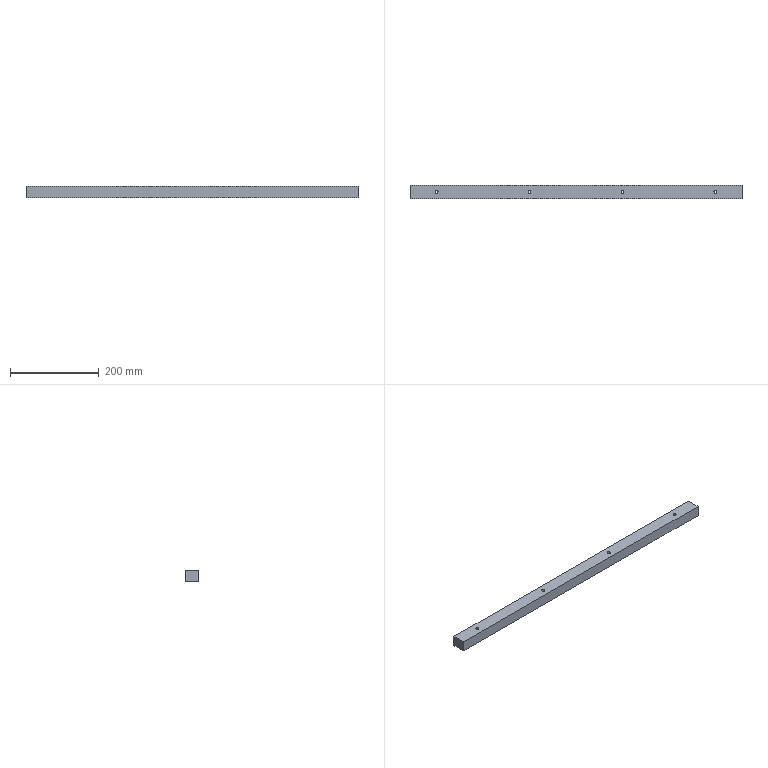Component | SolidWorks | DC-Motor-112-1 | 1 solid | 26 faces | box 750 x 30 x 25 mm | volume 557522 mm3 | cylinder 16 | plane 10 | commonest cylinder face diameters 11 x8 6.6 x8
build123d program:
from build123d import *

# Parameters (mm, degrees)
SKETCH1_W                                       = 750
SKETCH1_H                                       = 30
BOSS_EXTRUDE1_DEPTH                             = 12.5
M6_HEX_SOCKET_HEAD_CAP_SCREW_CBORE1_D           = 6.6
M6_HEX_SOCKET_HEAD_CAP_SCREW_CBORE1_CBORE_D     = 11
M6_HEX_SOCKET_HEAD_CAP_SCREW_CBORE1_CBORE_DEPTH = 6.4


with BuildPart() as part:
    # Sketch1 → Boss-Extrude1 (new, symmetric)
    with BuildSketch(Plane.XY):
        Rectangle(SKETCH1_W, SKETCH1_H)
    extrude(amount=BOSS_EXTRUDE1_DEPTH, both=True)

    # M6 Hex Socket Head Cap Screw CBORE1 (through all)
    with Locations(Plane.XY.offset(12.5)):
        with Locations((-315, 0), (-105, 0), (105, 0), (315, 0)):
            CounterBoreHole(M6_HEX_SOCKET_HEAD_CAP_SCREW_CBORE1_D / 2, M6_HEX_SOCKET_HEAD_CAP_SCREW_CBORE1_CBORE_D / 2, M6_HEX_SOCKET_HEAD_CAP_SCREW_CBORE1_CBORE_DEPTH)


solid = part.part

# Placed as in the assembly
solid = solid.moved(Location((177.208, 371.801, -438.5), (180, 0, 0)))
STEP:
#1=COLOUR_RGB('',0.7922,0.8196,0.9333);
#2=FILL_AREA_STYLE_COLOUR('',#1);
#3=FILL_AREA_STYLE('',(#2));
#4=SURFACE_STYLE_FILL_AREA(#3);
#5=SURFACE_SIDE_STYLE('',(#4));
#6=SURFACE_STYLE_USAGE(.BOTH.,#5);
#7=PRESENTATION_STYLE_ASSIGNMENT((#6));
#8=CARTESIAN_POINT('',(19.595,14.638,-17.504));
#9=VERTEX_POINT('',#8);
#10=CARTESIAN_POINT('',(19.162,14.638,-17.504));
#11=VERTEX_POINT('',#10);
#12=CARTESIAN_POINT('',(19.378,14.638,-17.504));
#13=DIRECTION('',(0.,0.,-1.));
#14=DIRECTION('',(-1.,0.,0.));
#15=AXIS2_PLACEMENT_3D('',#12,#13,#14);
#16=CIRCLE('',#15,0.2165);
#17=EDGE_CURVE('',#9,#11,#16,.T.);
#18=ORIENTED_EDGE('',*,*,#17,.F.);
#19=CARTESIAN_POINT('',(19.595,14.638,-17.756));
#20=VERTEX_POINT('',#19);
#21=CARTESIAN_POINT('',(19.595,14.638,-17.756));
#22=DIRECTION('',(0.,0.,-1.));
#23=VECTOR('',#22,39.37);
#24=LINE('',#21,#23);
#25=EDGE_CURVE('',#9,#20,#24,.T.);
#26=ORIENTED_EDGE('',*,*,#25,.T.);
#27=CARTESIAN_POINT('',(19.162,14.638,-17.756));
#28=VERTEX_POINT('',#27);
#29=CARTESIAN_POINT('',(19.378,14.638,-17.756));
#30=DIRECTION('',(0.,0.,-1.));
#31=DIRECTION('',(-1.,0.,0.));
#32=AXIS2_PLACEMENT_3D('',#29,#30,#31);
#33=CIRCLE('',#32,0.2165);
#34=EDGE_CURVE('',#20,#28,#33,.T.);
#35=ORIENTED_EDGE('',*,*,#34,.T.);
#36=CARTESIAN_POINT('',(19.162,14.638,-17.756));
#37=DIRECTION('',(0.,0.,-1.));
#38=VECTOR('',#37,39.37);
#39=LINE('',#36,#38);
#40=EDGE_CURVE('',#11,#28,#39,.T.);
#41=ORIENTED_EDGE('',*,*,#40,.F.);
#42=EDGE_LOOP('',(#18,#26,#35,#41));
#43=FACE_OUTER_BOUND('',#42,.T.);
#44=CARTESIAN_POINT('',(19.378,14.638,-17.756));
#45=DIRECTION('',(0.,0.,-1.));
#46=DIRECTION('',(-1.,0.,0.));
#47=AXIS2_PLACEMENT_3D('',#44,#45,#46);
#48=CYLINDRICAL_SURFACE('',#47,0.2165);
#49=ADVANCED_FACE('',(#43),#48,.F.);
#50=CARTESIAN_POINT('',(19.508,14.638,-16.772));
#51=VERTEX_POINT('',#50);
#52=CARTESIAN_POINT('',(19.248,14.638,-16.772));
#53=VERTEX_POINT('',#52);
#54=CARTESIAN_POINT('',(19.378,14.638,-16.772));
#55=DIRECTION('',(0.,0.,-1.));
#56=DIRECTION('',(-1.,0.,0.));
#57=AXIS2_PLACEMENT_3D('',#54,#55,#56);
#58=CIRCLE('',#57,0.1299);
#59=EDGE_CURVE('',#51,#53,#58,.T.);
#60=ORIENTED_EDGE('',*,*,#59,.F.);
#61=CARTESIAN_POINT('',(19.508,14.638,-17.504));
#62=VERTEX_POINT('',#61);
#63=CARTESIAN_POINT('',(19.508,14.638,-17.756));
#64=DIRECTION('',(0.,0.,-1.));
#65=VECTOR('',#64,39.37);
#66=LINE('',#63,#65);
#67=EDGE_CURVE('',#51,#62,#66,.T.);
#68=ORIENTED_EDGE('',*,*,#67,.T.);
#69=CARTESIAN_POINT('',(19.248,14.638,-17.504));
#70=VERTEX_POINT('',#69);
#71=CARTESIAN_POINT('',(19.378,14.638,-17.504));
#72=DIRECTION('',(0.,0.,-1.));
#73=DIRECTION('',(-1.,0.,0.));
#74=AXIS2_PLACEMENT_3D('',#71,#72,#73);
#75=CIRCLE('',#74,0.1299);
#76=EDGE_CURVE('',#62,#70,#75,.T.);
#77=ORIENTED_EDGE('',*,*,#76,.T.);
#78=CARTESIAN_POINT('',(19.248,14.638,-17.756));
#79=DIRECTION('',(0.,0.,-1.));
#80=VECTOR('',#79,39.37);
#81=LINE('',#78,#80);
#82=EDGE_CURVE('',#53,#70,#81,.T.);
#83=ORIENTED_EDGE('',*,*,#82,.F.);
#84=EDGE_LOOP('',(#60,#68,#77,#83));
#85=FACE_OUTER_BOUND('',#84,.T.);
#86=CARTESIAN_POINT('',(19.378,14.638,-17.756));
#87=DIRECTION('',(0.,0.,-1.));
#88=DIRECTION('',(-1.,0.,0.));
#89=AXIS2_PLACEMENT_3D('',#86,#87,#88);
#90=CYLINDRICAL_SURFACE('',#89,0.1299);
#91=ADVANCED_FACE('',(#85),#90,.F.);
#92=CARTESIAN_POINT('',(11.327,14.638,-17.504));
#93=VERTEX_POINT('',#92);
#94=CARTESIAN_POINT('',(10.894,14.638,-17.504));
#95=VERTEX_POINT('',#94);
#96=CARTESIAN_POINT('',(11.111,14.638,-17.504));
#97=DIRECTION('',(0.,0.,-1.));
#98=DIRECTION('',(-1.,0.,0.));
#99=AXIS2_PLACEMENT_3D('',#96,#97,#98);
#100=CIRCLE('',#99,0.2165);
#101=EDGE_CURVE('',#93,#95,#100,.T.);
#102=ORIENTED_EDGE('',*,*,#101,.F.);
#103=CARTESIAN_POINT('',(11.327,14.638,-17.756));
#104=VERTEX_POINT('',#103);
#105=CARTESIAN_POINT('',(11.327,14.638,-17.756));
#106=DIRECTION('',(0.,0.,-1.));
#107=VECTOR('',#106,39.37);
#108=LINE('',#105,#107);
#109=EDGE_CURVE('',#93,#104,#108,.T.);
#110=ORIENTED_EDGE('',*,*,#109,.T.);
#111=CARTESIAN_POINT('',(10.894,14.638,-17.756));
#112=VERTEX_POINT('',#111);
#113=CARTESIAN_POINT('',(11.111,14.638,-17.756));
#114=DIRECTION('',(0.,0.,-1.));
#115=DIRECTION('',(-1.,0.,0.));
#116=AXIS2_PLACEMENT_3D('',#113,#114,#115);
#117=CIRCLE('',#116,0.2165);
#118=EDGE_CURVE('',#104,#112,#117,.T.);
#119=ORIENTED_EDGE('',*,*,#118,.T.);
#120=CARTESIAN_POINT('',(10.894,14.638,-17.756));
#121=DIRECTION('',(0.,0.,-1.));
#122=VECTOR('',#121,39.37);
#123=LINE('',#120,#122);
#124=EDGE_CURVE('',#95,#112,#123,.T.);
#125=ORIENTED_EDGE('',*,*,#124,.F.);
#126=EDGE_LOOP('',(#102,#110,#119,#125));
#127=FACE_OUTER_BOUND('',#126,.T.);
#128=CARTESIAN_POINT('',(11.111,14.638,-17.756));
#129=DIRECTION('',(0.,0.,-1.));
#130=DIRECTION('',(-1.,0.,0.));
#131=AXIS2_PLACEMENT_3D('',#128,#129,#130);
#132=CYLINDRICAL_SURFACE('',#131,0.2165);
#133=ADVANCED_FACE('',(#127),#132,.F.);
#134=CARTESIAN_POINT('',(11.24,14.638,-16.772));
#135=VERTEX_POINT('',#134);
#136=CARTESIAN_POINT('',(10.981,14.638,-16.772));
#137=VERTEX_POINT('',#136);
#138=CARTESIAN_POINT('',(11.111,14.638,-16.772));
#139=DIRECTION('',(0.,0.,-1.));
#140=DIRECTION('',(-1.,0.,0.));
#141=AXIS2_PLACEMENT_3D('',#138,#139,#140);
#142=CIRCLE('',#141,0.1299);
#143=EDGE_CURVE('',#135,#137,#142,.T.);
#144=ORIENTED_EDGE('',*,*,#143,.F.);
#145=CARTESIAN_POINT('',(11.24,14.638,-17.504));
#146=VERTEX_POINT('',#145);
#147=CARTESIAN_POINT('',(11.24,14.638,-17.756));
#148=DIRECTION('',(0.,0.,-1.));
#149=VECTOR('',#148,39.37);
#150=LINE('',#147,#149);
#151=EDGE_CURVE('',#135,#146,#150,.T.);
#152=ORIENTED_EDGE('',*,*,#151,.T.);
#153=CARTESIAN_POINT('',(10.981,14.638,-17.504));
#154=VERTEX_POINT('',#153);
#155=CARTESIAN_POINT('',(11.111,14.638,-17.504));
#156=DIRECTION('',(0.,0.,-1.));
#157=DIRECTION('',(-1.,0.,0.));
#158=AXIS2_PLACEMENT_3D('',#155,#156,#157);
#159=CIRCLE('',#158,0.1299);
#160=EDGE_CURVE('',#146,#154,#159,.T.);
#161=ORIENTED_EDGE('',*,*,#160,.T.);
#162=CARTESIAN_POINT('',(10.981,14.638,-17.756));
#163=DIRECTION('',(0.,0.,-1.));
#164=VECTOR('',#163,39.37);
#165=LINE('',#162,#164);
#166=EDGE_CURVE('',#137,#154,#165,.T.);
#167=ORIENTED_EDGE('',*,*,#166,.F.);
#168=EDGE_LOOP('',(#144,#152,#161,#167));
#169=FACE_OUTER_BOUND('',#168,.T.);
#170=CARTESIAN_POINT('',(11.111,14.638,-17.756));
#171=DIRECTION('',(0.,0.,-1.));
#172=DIRECTION('',(-1.,0.,0.));
#173=AXIS2_PLACEMENT_3D('',#170,#171,#172);
#174=CYLINDRICAL_SURFACE('',#173,0.1299);
#175=ADVANCED_FACE('',(#169),#174,.F.);
#176=CARTESIAN_POINT('',(3.059,14.638,-17.504));
#177=VERTEX_POINT('',#176);
#178=CARTESIAN_POINT('',(2.626,14.638,-17.504));
#179=VERTEX_POINT('',#178);
#180=CARTESIAN_POINT('',(2.843,14.638,-17.504));
#181=DIRECTION('',(0.,0.,-1.));
#182=DIRECTION('',(-1.,0.,0.));
#183=AXIS2_PLACEMENT_3D('',#180,#181,#182);
#184=CIRCLE('',#183,0.2165);
#185=EDGE_CURVE('',#177,#179,#184,.T.);
#186=ORIENTED_EDGE('',*,*,#185,.F.);
#187=CARTESIAN_POINT('',(3.059,14.638,-17.756));
#188=VERTEX_POINT('',#187);
#189=CARTESIAN_POINT('',(3.059,14.638,-17.756));
#190=DIRECTION('',(0.,0.,-1.));
#191=VECTOR('',#190,39.37);
#192=LINE('',#189,#191);
#193=EDGE_CURVE('',#177,#188,#192,.T.);
#194=ORIENTED_EDGE('',*,*,#193,.T.);
#195=CARTESIAN_POINT('',(2.626,14.638,-17.756));
#196=VERTEX_POINT('',#195);
#197=CARTESIAN_POINT('',(2.843,14.638,-17.756));
#198=DIRECTION('',(0.,0.,-1.));
#199=DIRECTION('',(-1.,0.,0.));
#200=AXIS2_PLACEMENT_3D('',#197,#198,#199);
#201=CIRCLE('',#200,0.2165);
#202=EDGE_CURVE('',#188,#196,#201,.T.);
#203=ORIENTED_EDGE('',*,*,#202,.T.);
#204=CARTESIAN_POINT('',(2.626,14.638,-17.756));
#205=DIRECTION('',(0.,0.,-1.));
#206=VECTOR('',#205,39.37);
#207=LINE('',#204,#206);
#208=EDGE_CURVE('',#179,#196,#207,.T.);
#209=ORIENTED_EDGE('',*,*,#208,.F.);
#210=EDGE_LOOP('',(#186,#194,#203,#209));
#211=FACE_OUTER_BOUND('',#210,.T.);
#212=CARTESIAN_POINT('',(2.843,14.638,-17.756));
#213=DIRECTION('',(0.,0.,-1.));
#214=DIRECTION('',(-1.,0.,0.));
#215=AXIS2_PLACEMENT_3D('',#212,#213,#214);
#216=CYLINDRICAL_SURFACE('',#215,0.2165);
#217=ADVANCED_FACE('',(#211),#216,.F.);
#218=CARTESIAN_POINT('',(2.973,14.638,-16.772));
#219=VERTEX_POINT('',#218);
#220=CARTESIAN_POINT('',(2.713,14.638,-16.772));
#221=VERTEX_POINT('',#220);
#222=CARTESIAN_POINT('',(2.843,14.638,-16.772));
#223=DIRECTION('',(0.,0.,-1.));
#224=DIRECTION('',(-1.,0.,0.));
#225=AXIS2_PLACEMENT_3D('',#222,#223,#224);
#226=CIRCLE('',#225,0.1299);
#227=EDGE_CURVE('',#219,#221,#226,.T.);
#228=ORIENTED_EDGE('',*,*,#227,.F.);
#229=CARTESIAN_POINT('',(2.973,14.638,-17.504));
#230=VERTEX_POINT('',#229);
#231=CARTESIAN_POINT('',(2.973,14.638,-17.756));
#232=DIRECTION('',(0.,0.,-1.));
#233=VECTOR('',#232,39.37);
#234=LINE('',#231,#233);
#235=EDGE_CURVE('',#219,#230,#234,.T.);
#236=ORIENTED_EDGE('',*,*,#235,.T.);
#237=CARTESIAN_POINT('',(2.713,14.638,-17.504));
#238=VERTEX_POINT('',#237);
#239=CARTESIAN_POINT('',(2.843,14.638,-17.504));
#240=DIRECTION('',(0.,0.,-1.));
#241=DIRECTION('',(-1.,0.,0.));
#242=AXIS2_PLACEMENT_3D('',#239,#240,#241);
#243=CIRCLE('',#242,0.1299);
#244=EDGE_CURVE('',#230,#238,#243,.T.);
#245=ORIENTED_EDGE('',*,*,#244,.T.);
#246=CARTESIAN_POINT('',(2.713,14.638,-17.756));
#247=DIRECTION('',(0.,0.,-1.));
#248=VECTOR('',#247,39.37);
#249=LINE('',#246,#248);
#250=EDGE_CURVE('',#221,#238,#249,.T.);
#251=ORIENTED_EDGE('',*,*,#250,.F.);
#252=EDGE_LOOP('',(#228,#236,#245,#251));
#253=FACE_OUTER_BOUND('',#252,.T.);
#254=CARTESIAN_POINT('',(2.843,14.638,-17.756));
#255=DIRECTION('',(0.,0.,-1.));
#256=DIRECTION('',(-1.,0.,0.));
#257=AXIS2_PLACEMENT_3D('',#254,#255,#256);
#258=CYLINDRICAL_SURFACE('',#257,0.1299);
#259=ADVANCED_FACE('',(#253),#258,.F.);
#260=CARTESIAN_POINT('',(-5.208,14.638,-17.504));
#261=VERTEX_POINT('',#260);
#262=CARTESIAN_POINT('',(-5.641,14.638,-17.504));
#263=VERTEX_POINT('',#262);
#264=CARTESIAN_POINT('',(-5.425,14.638,-17.504));
#265=DIRECTION('',(0.,0.,-1.));
#266=DIRECTION('',(-1.,0.,0.));
#267=AXIS2_PLACEMENT_3D('',#264,#265,#266);
#268=CIRCLE('',#267,0.2165);
#269=EDGE_CURVE('',#261,#263,#268,.T.);
#270=ORIENTED_EDGE('',*,*,#269,.F.);
#271=CARTESIAN_POINT('',(-5.208,14.638,-17.756));
#272=VERTEX_POINT('',#271);
#273=CARTESIAN_POINT('',(-5.208,14.638,-17.756));
#274=DIRECTION('',(0.,0.,-1.));
#275=VECTOR('',#274,39.37);
#276=LINE('',#273,#275);
#277=EDGE_CURVE('',#261,#272,#276,.T.);
#278=ORIENTED_EDGE('',*,*,#277,.T.);
#279=CARTESIAN_POINT('',(-5.641,14.638,-17.756));
#280=VERTEX_POINT('',#279);
#281=CARTESIAN_POINT('',(-5.425,14.638,-17.756));
#282=DIRECTION('',(0.,0.,-1.));
#283=DIRECTION('',(-1.,0.,0.));
#284=AXIS2_PLACEMENT_3D('',#281,#282,#283);
#285=CIRCLE('',#284,0.2165);
#286=EDGE_CURVE('',#272,#280,#285,.T.);
#287=ORIENTED_EDGE('',*,*,#286,.T.);
#288=CARTESIAN_POINT('',(-5.641,14.638,-17.756));
#289=DIRECTION('',(0.,0.,-1.));
#290=VECTOR('',#289,39.37);
#291=LINE('',#288,#290);
#292=EDGE_CURVE('',#263,#280,#291,.T.);
#293=ORIENTED_EDGE('',*,*,#292,.F.);
#294=EDGE_LOOP('',(#270,#278,#287,#293));
#295=FACE_OUTER_BOUND('',#294,.T.);
#296=CARTESIAN_POINT('',(-5.425,14.638,-17.756));
#297=DIRECTION('',(0.,0.,-1.));
#298=DIRECTION('',(-1.,0.,0.));
#299=AXIS2_PLACEMENT_3D('',#296,#297,#298);
#300=CYLINDRICAL_SURFACE('',#299,0.2165);
#301=ADVANCED_FACE('',(#295),#300,.F.);
#302=CARTESIAN_POINT('',(-5.295,14.638,-16.772));
#303=VERTEX_POINT('',#302);
#304=CARTESIAN_POINT('',(-5.555,14.638,-16.772));
#305=VERTEX_POINT('',#304);
#306=CARTESIAN_POINT('',(-5.425,14.638,-16.772));
#307=DIRECTION('',(0.,0.,-1.));
#308=DIRECTION('',(-1.,0.,0.));
#309=AXIS2_PLACEMENT_3D('',#306,#307,#308);
#310=CIRCLE('',#309,0.1299);
#311=EDGE_CURVE('',#303,#305,#310,.T.);
#312=ORIENTED_EDGE('',*,*,#311,.F.);
#313=CARTESIAN_POINT('',(-5.295,14.638,-17.504));
#314=VERTEX_POINT('',#313);
#315=CARTESIAN_POINT('',(-5.295,14.638,-17.756));
#316=DIRECTION('',(0.,0.,-1.));
#317=VECTOR('',#316,39.37);
#318=LINE('',#315,#317);
#319=EDGE_CURVE('',#303,#314,#318,.T.);
#320=ORIENTED_EDGE('',*,*,#319,.T.);
#321=CARTESIAN_POINT('',(-5.555,14.638,-17.504));
#322=VERTEX_POINT('',#321);
#323=CARTESIAN_POINT('',(-5.425,14.638,-17.504));
#324=DIRECTION('',(0.,0.,-1.));
#325=DIRECTION('',(-1.,0.,0.));
#326=AXIS2_PLACEMENT_3D('',#323,#324,#325);
#327=CIRCLE('',#326,0.1299);
#328=EDGE_CURVE('',#314,#322,#327,.T.);
#329=ORIENTED_EDGE('',*,*,#328,.T.);
#330=CARTESIAN_POINT('',(-5.555,14.638,-17.756));
#331=DIRECTION('',(0.,0.,-1.));
#332=VECTOR('',#331,39.37);
#333=LINE('',#330,#332);
#334=EDGE_CURVE('',#305,#322,#333,.T.);
#335=ORIENTED_EDGE('',*,*,#334,.F.);
#336=EDGE_LOOP('',(#312,#320,#329,#335));
#337=FACE_OUTER_BOUND('',#336,.T.);
#338=CARTESIAN_POINT('',(-5.425,14.638,-17.756));
#339=DIRECTION('',(0.,0.,-1.));
#340=DIRECTION('',(-1.,0.,0.));
#341=AXIS2_PLACEMENT_3D('',#338,#339,#340);
#342=CYLINDRICAL_SURFACE('',#341,0.1299);
#343=ADVANCED_FACE('',(#337),#342,.F.);
#344=CARTESIAN_POINT('',(21.74,15.228,-16.772));
#345=VERTEX_POINT('',#344);
#346=CARTESIAN_POINT('',(21.74,14.047,-16.772));
#347=VERTEX_POINT('',#346);
#348=CARTESIAN_POINT('',(21.74,14.047,-16.772));
#349=DIRECTION('',(0.,-1.,0.));
#350=VECTOR('',#349,39.37);
#351=LINE('',#348,#350);
#352=EDGE_CURVE('',#345,#347,#351,.T.);
#353=ORIENTED_EDGE('',*,*,#352,.T.);
#354=CARTESIAN_POINT('',(21.74,14.047,-17.756));
#355=VERTEX_POINT('',#354);
#356=CARTESIAN_POINT('',(21.74,14.047,-17.756));
#357=DIRECTION('',(0.,0.,1.));
#358=VECTOR('',#357,39.37);
#359=LINE('',#356,#358);
#360=EDGE_CURVE('',#355,#347,#359,.T.);
#361=ORIENTED_EDGE('',*,*,#360,.F.);
#362=CARTESIAN_POINT('',(21.74,15.228,-17.756));
#363=VERTEX_POINT('',#362);
#364=CARTESIAN_POINT('',(21.74,14.047,-17.756));
#365=DIRECTION('',(0.,-1.,0.));
#366=VECTOR('',#365,39.37);
#367=LINE('',#364,#366);
#368=EDGE_CURVE('',#363,#355,#367,.T.);
#369=ORIENTED_EDGE('',*,*,#368,.F.);
#370=CARTESIAN_POINT('',(21.74,15.228,-17.756));
#371=DIRECTION('',(0.,0.,1.));
#372=VECTOR('',#371,39.37);
#373=LINE('',#370,#372);
#374=EDGE_CURVE('',#363,#345,#373,.T.);
#375=ORIENTED_EDGE('',*,*,#374,.T.);
#376=EDGE_LOOP('',(#353,#361,#369,#375));
#377=FACE_OUTER_BOUND('',#376,.T.);
#378=CARTESIAN_POINT('',(21.74,14.047,-17.756));
#379=DIRECTION('',(-1.,-0.,0.));
#380=DIRECTION('',(0.,0.,1.));
#381=AXIS2_PLACEMENT_3D('',#378,#379,#380);
#382=PLANE('',#381);
#383=ADVANCED_FACE('',(#377),#382,.F.);
#384=CARTESIAN_POINT('',(-7.787,14.047,-16.772));
#385=VERTEX_POINT('',#384);
#386=CARTESIAN_POINT('',(-7.787,14.047,-16.772));
#387=DIRECTION('',(-1.,-0.,0.));
#388=VECTOR('',#387,39.37);
#389=LINE('',#386,#388);
#390=EDGE_CURVE('',#347,#385,#389,.T.);
#391=ORIENTED_EDGE('',*,*,#390,.T.);
#392=CARTESIAN_POINT('',(-7.787,14.047,-17.756));
#393=VERTEX_POINT('',#392);
#394=CARTESIAN_POINT('',(-7.787,14.047,-17.756));
#395=DIRECTION('',(0.,0.,1.));
#396=VECTOR('',#395,39.37);
#397=LINE('',#394,#396);
#398=EDGE_CURVE('',#393,#385,#397,.T.);
#399=ORIENTED_EDGE('',*,*,#398,.F.);
#400=CARTESIAN_POINT('',(-7.787,14.047,-17.756));
#401=DIRECTION('',(-1.,-0.,0.));
#402=VECTOR('',#401,39.37);
#403=LINE('',#400,#402);
#404=EDGE_CURVE('',#355,#393,#403,.T.);
#405=ORIENTED_EDGE('',*,*,#404,.F.);
#406=ORIENTED_EDGE('',*,*,#360,.T.);
#407=EDGE_LOOP('',(#391,#399,#405,#406));
#408=FACE_OUTER_BOUND('',#407,.T.);
#409=CARTESIAN_POINT('',(-7.787,14.047,-17.756));
#410=DIRECTION('',(-0.,1.,0.));
#411=DIRECTION('',(1.,0.,0.));
#412=AXIS2_PLACEMENT_3D('',#409,#410,#411);
#413=PLANE('',#412);
#414=ADVANCED_FACE('',(#408),#413,.F.);
#415=CARTESIAN_POINT('',(-7.787,15.228,-16.772));
#416=VERTEX_POINT('',#415);
#417=CARTESIAN_POINT('',(-7.787,14.047,-16.772));
#418=DIRECTION('',(-0.,1.,0.));
#419=VECTOR('',#418,39.37);
#420=LINE('',#417,#419);
#421=EDGE_CURVE('',#385,#416,#420,.T.);
#422=ORIENTED_EDGE('',*,*,#421,.T.);
#423=CARTESIAN_POINT('',(-7.787,15.228,-17.756));
#424=VERTEX_POINT('',#423);
#425=CARTESIAN_POINT('',(-7.787,15.228,-17.756));
#426=DIRECTION('',(0.,0.,1.));
#427=VECTOR('',#426,39.37);
#428=LINE('',#425,#427);
#429=EDGE_CURVE('',#424,#416,#428,.T.);
#430=ORIENTED_EDGE('',*,*,#429,.F.);
#431=CARTESIAN_POINT('',(-7.787,14.047,-17.756));
#432=DIRECTION('',(-0.,1.,0.));
#433=VECTOR('',#432,39.37);
#434=LINE('',#431,#433);
#435=EDGE_CURVE('',#393,#424,#434,.T.);
#436=ORIENTED_EDGE('',*,*,#435,.F.);
#437=ORIENTED_EDGE('',*,*,#398,.T.);
#438=EDGE_LOOP('',(#422,#430,#436,#437));
#439=FACE_OUTER_BOUND('',#438,.T.);
#440=CARTESIAN_POINT('',(-7.787,14.047,-17.756));
#441=DIRECTION('',(1.,0.,0.));
#442=DIRECTION('',(0.,0.,-1.));
#443=AXIS2_PLACEMENT_3D('',#440,#441,#442);
#444=PLANE('',#443);
#445=ADVANCED_FACE('',(#439),#444,.F.);
#446=CARTESIAN_POINT('',(-7.787,15.228,-16.772));
#447=DIRECTION('',(1.,0.,0.));
#448=VECTOR('',#447,39.37);
#449=LINE('',#446,#448);
#450=EDGE_CURVE('',#416,#345,#449,.T.);
#451=ORIENTED_EDGE('',*,*,#450,.T.);
#452=ORIENTED_EDGE('',*,*,#374,.F.);
#453=CARTESIAN_POINT('',(-7.787,15.228,-17.756));
#454=DIRECTION('',(1.,0.,0.));
#455=VECTOR('',#454,39.37);
#456=LINE('',#453,#455);
#457=EDGE_CURVE('',#424,#363,#456,.T.);
#458=ORIENTED_EDGE('',*,*,#457,.F.);
#459=ORIENTED_EDGE('',*,*,#429,.T.);
#460=EDGE_LOOP('',(#451,#452,#458,#459));
#461=FACE_OUTER_BOUND('',#460,.T.);
#462=CARTESIAN_POINT('',(-7.787,15.228,-17.756));
#463=DIRECTION('',(0.,-1.,0.));
#464=DIRECTION('',(-1.,-0.,0.));
#465=AXIS2_PLACEMENT_3D('',#462,#463,#464);
#466=PLANE('',#465);
#467=ADVANCED_FACE('',(#461),#466,.F.);
#468=CARTESIAN_POINT('',(19.378,14.638,-17.756));
#469=DIRECTION('',(0.,0.,-1.));
#470=DIRECTION('',(-1.,0.,0.));
#471=AXIS2_PLACEMENT_3D('',#468,#469,#470);
#472=CIRCLE('',#471,0.2165);
#473=EDGE_CURVE('',#28,#20,#472,.T.);
#474=ORIENTED_EDGE('',*,*,#473,.F.);
#475=ORIENTED_EDGE('',*,*,#34,.F.);
#476=EDGE_LOOP('',(#474,#475));
#477=FACE_BOUND('',#476,.T.);
#478=CARTESIAN_POINT('',(11.111,14.638,-17.756));
#479=DIRECTION('',(0.,0.,-1.));
#480=DIRECTION('',(-1.,0.,0.));
#481=AXIS2_PLACEMENT_3D('',#478,#479,#480);
#482=CIRCLE('',#481,0.2165);
#483=EDGE_CURVE('',#112,#104,#482,.T.);
#484=ORIENTED_EDGE('',*,*,#483,.F.);
#485=ORIENTED_EDGE('',*,*,#118,.F.);
#486=EDGE_LOOP('',(#484,#485));
#487=FACE_BOUND('',#486,.T.);
#488=CARTESIAN_POINT('',(2.843,14.638,-17.756));
#489=DIRECTION('',(0.,0.,-1.));
#490=DIRECTION('',(-1.,0.,0.));
#491=AXIS2_PLACEMENT_3D('',#488,#489,#490);
#492=CIRCLE('',#491,0.2165);
#493=EDGE_CURVE('',#196,#188,#492,.T.);
#494=ORIENTED_EDGE('',*,*,#493,.F.);
#495=ORIENTED_EDGE('',*,*,#202,.F.);
#496=EDGE_LOOP('',(#494,#495));
#497=FACE_BOUND('',#496,.T.);
#498=CARTESIAN_POINT('',(-5.425,14.638,-17.756));
#499=DIRECTION('',(0.,0.,-1.));
#500=DIRECTION('',(-1.,0.,0.));
#501=AXIS2_PLACEMENT_3D('',#498,#499,#500);
#502=CIRCLE('',#501,0.2165);
#503=EDGE_CURVE('',#280,#272,#502,.T.);
#504=ORIENTED_EDGE('',*,*,#503,.F.);
#505=ORIENTED_EDGE('',*,*,#286,.F.);
#506=EDGE_LOOP('',(#504,#505));
#507=FACE_BOUND('',#506,.T.);
#508=ORIENTED_EDGE('',*,*,#368,.T.);
#509=ORIENTED_EDGE('',*,*,#404,.T.);
#510=ORIENTED_EDGE('',*,*,#435,.T.);
#511=ORIENTED_EDGE('',*,*,#457,.T.);
#512=EDGE_LOOP('',(#508,#509,#510,#511));
#513=FACE_OUTER_BOUND('',#512,.T.);
#514=CARTESIAN_POINT('',(6.977,14.638,-17.756));
#515=DIRECTION('',(0.,0.,-1.));
#516=DIRECTION('',(-1.,-0.,0.));
#517=AXIS2_PLACEMENT_3D('',#514,#515,#516);
#518=PLANE('',#517);
#519=ADVANCED_FACE('',(#477,#487,#497,#507,#513),#518,.T.);
#520=CARTESIAN_POINT('',(19.378,14.638,-16.772));
#521=DIRECTION('',(0.,0.,-1.));
#522=DIRECTION('',(-1.,0.,0.));
#523=AXIS2_PLACEMENT_3D('',#520,#521,#522);
#524=CIRCLE('',#523,0.1299);
#525=EDGE_CURVE('',#53,#51,#524,.T.);
#526=ORIENTED_EDGE('',*,*,#525,.T.);
#527=ORIENTED_EDGE('',*,*,#59,.T.);
#528=EDGE_LOOP('',(#526,#527));
#529=FACE_BOUND('',#528,.T.);
#530=CARTESIAN_POINT('',(11.111,14.638,-16.772));
#531=DIRECTION('',(0.,0.,-1.));
#532=DIRECTION('',(-1.,0.,0.));
#533=AXIS2_PLACEMENT_3D('',#530,#531,#532);
#534=CIRCLE('',#533,0.1299);
#535=EDGE_CURVE('',#137,#135,#534,.T.);
#536=ORIENTED_EDGE('',*,*,#535,.T.);
#537=ORIENTED_EDGE('',*,*,#143,.T.);
#538=EDGE_LOOP('',(#536,#537));
#539=FACE_BOUND('',#538,.T.);
#540=CARTESIAN_POINT('',(2.843,14.638,-16.772));
#541=DIRECTION('',(0.,0.,-1.));
#542=DIRECTION('',(-1.,0.,0.));
#543=AXIS2_PLACEMENT_3D('',#540,#541,#542);
#544=CIRCLE('',#543,0.1299);
#545=EDGE_CURVE('',#221,#219,#544,.T.);
#546=ORIENTED_EDGE('',*,*,#545,.T.);
#547=ORIENTED_EDGE('',*,*,#227,.T.);
#548=EDGE_LOOP('',(#546,#547));
#549=FACE_BOUND('',#548,.T.);
#550=CARTESIAN_POINT('',(-5.425,14.638,-16.772));
#551=DIRECTION('',(0.,0.,-1.));
#552=DIRECTION('',(-1.,0.,0.));
#553=AXIS2_PLACEMENT_3D('',#550,#551,#552);
#554=CIRCLE('',#553,0.1299);
#555=EDGE_CURVE('',#305,#303,#554,.T.);
#556=ORIENTED_EDGE('',*,*,#555,.T.);
#557=ORIENTED_EDGE('',*,*,#311,.T.);
#558=EDGE_LOOP('',(#556,#557));
#559=FACE_BOUND('',#558,.T.);
#560=ORIENTED_EDGE('',*,*,#352,.F.);
#561=ORIENTED_EDGE('',*,*,#450,.F.);
#562=ORIENTED_EDGE('',*,*,#421,.F.);
#563=ORIENTED_EDGE('',*,*,#390,.F.);
#564=EDGE_LOOP('',(#560,#561,#562,#563));
#565=FACE_OUTER_BOUND('',#564,.T.);
#566=CARTESIAN_POINT('',(6.977,14.638,-16.772));
#567=DIRECTION('',(0.,0.,-1.));
#568=DIRECTION('',(-1.,-0.,0.));
#569=AXIS2_PLACEMENT_3D('',#566,#567,#568);
#570=PLANE('',#569);
#571=ADVANCED_FACE('',(#529,#539,#549,#559,#565),#570,.F.);
#572=ORIENTED_EDGE('',*,*,#319,.F.);
#573=ORIENTED_EDGE('',*,*,#555,.F.);
#574=ORIENTED_EDGE('',*,*,#334,.T.);
#575=CARTESIAN_POINT('',(-5.425,14.638,-17.504));
#576=DIRECTION('',(0.,0.,-1.));
#577=DIRECTION('',(-1.,0.,0.));
#578=AXIS2_PLACEMENT_3D('',#575,#576,#577);
#579=CIRCLE('',#578,0.1299);
#580=EDGE_CURVE('',#322,#314,#579,.T.);
#581=ORIENTED_EDGE('',*,*,#580,.T.);
#582=EDGE_LOOP('',(#572,#573,#574,#581));
#583=FACE_OUTER_BOUND('',#582,.T.);
#584=CARTESIAN_POINT('',(-5.425,14.638,-17.756));
#585=DIRECTION('',(0.,0.,-1.));
#586=DIRECTION('',(-1.,0.,0.));
#587=AXIS2_PLACEMENT_3D('',#584,#585,#586);
#588=CYLINDRICAL_SURFACE('',#587,0.1299);
#589=ADVANCED_FACE('',(#583),#588,.F.);
#590=ORIENTED_EDGE('',*,*,#580,.F.);
#591=ORIENTED_EDGE('',*,*,#328,.F.);
#592=EDGE_LOOP('',(#590,#591));
#593=FACE_BOUND('',#592,.T.);
#594=CARTESIAN_POINT('',(-5.425,14.638,-17.504));
#595=DIRECTION('',(0.,0.,-1.));
#596=DIRECTION('',(-1.,0.,0.));
#597=AXIS2_PLACEMENT_3D('',#594,#595,#596);
#598=CIRCLE('',#597,0.2165);
#599=EDGE_CURVE('',#263,#261,#598,.T.);
#600=ORIENTED_EDGE('',*,*,#599,.T.);
#601=ORIENTED_EDGE('',*,*,#269,.T.);
#602=EDGE_LOOP('',(#600,#601));
#603=FACE_OUTER_BOUND('',#602,.T.);
#604=CARTESIAN_POINT('',(-5.555,14.638,-17.504));
#605=DIRECTION('',(0.,0.,1.));
#606=DIRECTION('',(1.,0.,0.));
#607=AXIS2_PLACEMENT_3D('',#604,#605,#606);
#608=PLANE('',#607);
#609=ADVANCED_FACE('',(#593,#603),#608,.F.);
#610=ORIENTED_EDGE('',*,*,#277,.F.);
#611=ORIENTED_EDGE('',*,*,#599,.F.);
#612=ORIENTED_EDGE('',*,*,#292,.T.);
#613=ORIENTED_EDGE('',*,*,#503,.T.);
#614=EDGE_LOOP('',(#610,#611,#612,#613));
#615=FACE_OUTER_BOUND('',#614,.T.);
#616=CARTESIAN_POINT('',(-5.425,14.638,-17.756));
#617=DIRECTION('',(0.,0.,-1.));
#618=DIRECTION('',(-1.,0.,0.));
#619=AXIS2_PLACEMENT_3D('',#616,#617,#618);
#620=CYLINDRICAL_SURFACE('',#619,0.2165);
#621=ADVANCED_FACE('',(#615),#620,.F.);
#622=ORIENTED_EDGE('',*,*,#235,.F.);
#623=ORIENTED_EDGE('',*,*,#545,.F.);
#624=ORIENTED_EDGE('',*,*,#250,.T.);
#625=CARTESIAN_POINT('',(2.843,14.638,-17.504));
#626=DIRECTION('',(0.,0.,-1.));
#627=DIRECTION('',(-1.,0.,0.));
#628=AXIS2_PLACEMENT_3D('',#625,#626,#627);
#629=CIRCLE('',#628,0.1299);
#630=EDGE_CURVE('',#238,#230,#629,.T.);
#631=ORIENTED_EDGE('',*,*,#630,.T.);
#632=EDGE_LOOP('',(#622,#623,#624,#631));
#633=FACE_OUTER_BOUND('',#632,.T.);
#634=CARTESIAN_POINT('',(2.843,14.638,-17.756));
#635=DIRECTION('',(0.,0.,-1.));
#636=DIRECTION('',(-1.,0.,0.));
#637=AXIS2_PLACEMENT_3D('',#634,#635,#636);
#638=CYLINDRICAL_SURFACE('',#637,0.1299);
#639=ADVANCED_FACE('',(#633),#638,.F.);
#640=ORIENTED_EDGE('',*,*,#630,.F.);
#641=ORIENTED_EDGE('',*,*,#244,.F.);
#642=EDGE_LOOP('',(#640,#641));
#643=FACE_BOUND('',#642,.T.);
#644=CARTESIAN_POINT('',(2.843,14.638,-17.504));
#645=DIRECTION('',(0.,0.,-1.));
#646=DIRECTION('',(-1.,0.,0.));
#647=AXIS2_PLACEMENT_3D('',#644,#645,#646);
#648=CIRCLE('',#647,0.2165);
#649=EDGE_CURVE('',#179,#177,#648,.T.);
#650=ORIENTED_EDGE('',*,*,#649,.T.);
#651=ORIENTED_EDGE('',*,*,#185,.T.);
#652=EDGE_LOOP('',(#650,#651));
#653=FACE_OUTER_BOUND('',#652,.T.);
#654=CARTESIAN_POINT('',(2.713,14.638,-17.504));
#655=DIRECTION('',(0.,0.,1.));
#656=DIRECTION('',(1.,0.,0.));
#657=AXIS2_PLACEMENT_3D('',#654,#655,#656);
#658=PLANE('',#657);
#659=ADVANCED_FACE('',(#643,#653),#658,.F.);
#660=ORIENTED_EDGE('',*,*,#193,.F.);
#661=ORIENTED_EDGE('',*,*,#649,.F.);
#662=ORIENTED_EDGE('',*,*,#208,.T.);
#663=ORIENTED_EDGE('',*,*,#493,.T.);
#664=EDGE_LOOP('',(#660,#661,#662,#663));
#665=FACE_OUTER_BOUND('',#664,.T.);
#666=CARTESIAN_POINT('',(2.843,14.638,-17.756));
#667=DIRECTION('',(0.,0.,-1.));
#668=DIRECTION('',(-1.,0.,0.));
#669=AXIS2_PLACEMENT_3D('',#666,#667,#668);
#670=CYLINDRICAL_SURFACE('',#669,0.2165);
#671=ADVANCED_FACE('',(#665),#670,.F.);
#672=ORIENTED_EDGE('',*,*,#151,.F.);
#673=ORIENTED_EDGE('',*,*,#535,.F.);
#674=ORIENTED_EDGE('',*,*,#166,.T.);
#675=CARTESIAN_POINT('',(11.111,14.638,-17.504));
#676=DIRECTION('',(0.,0.,-1.));
#677=DIRECTION('',(-1.,0.,0.));
#678=AXIS2_PLACEMENT_3D('',#675,#676,#677);
#679=CIRCLE('',#678,0.1299);
#680=EDGE_CURVE('',#154,#146,#679,.T.);
#681=ORIENTED_EDGE('',*,*,#680,.T.);
#682=EDGE_LOOP('',(#672,#673,#674,#681));
#683=FACE_OUTER_BOUND('',#682,.T.);
#684=CARTESIAN_POINT('',(11.111,14.638,-17.756));
#685=DIRECTION('',(0.,0.,-1.));
#686=DIRECTION('',(-1.,0.,0.));
#687=AXIS2_PLACEMENT_3D('',#684,#685,#686);
#688=CYLINDRICAL_SURFACE('',#687,0.1299);
#689=ADVANCED_FACE('',(#683),#688,.F.);
#690=ORIENTED_EDGE('',*,*,#680,.F.);
#691=ORIENTED_EDGE('',*,*,#160,.F.);
#692=EDGE_LOOP('',(#690,#691));
#693=FACE_BOUND('',#692,.T.);
#694=CARTESIAN_POINT('',(11.111,14.638,-17.504));
#695=DIRECTION('',(0.,0.,-1.));
#696=DIRECTION('',(-1.,0.,0.));
#697=AXIS2_PLACEMENT_3D('',#694,#695,#696);
#698=CIRCLE('',#697,0.2165);
#699=EDGE_CURVE('',#95,#93,#698,.T.);
#700=ORIENTED_EDGE('',*,*,#699,.T.);
#701=ORIENTED_EDGE('',*,*,#101,.T.);
#702=EDGE_LOOP('',(#700,#701));
#703=FACE_OUTER_BOUND('',#702,.T.);
#704=CARTESIAN_POINT('',(10.981,14.638,-17.504));
#705=DIRECTION('',(0.,0.,1.));
#706=DIRECTION('',(1.,0.,0.));
#707=AXIS2_PLACEMENT_3D('',#704,#705,#706);
#708=PLANE('',#707);
#709=ADVANCED_FACE('',(#693,#703),#708,.F.);
#710=ORIENTED_EDGE('',*,*,#109,.F.);
#711=ORIENTED_EDGE('',*,*,#699,.F.);
#712=ORIENTED_EDGE('',*,*,#124,.T.);
#713=ORIENTED_EDGE('',*,*,#483,.T.);
#714=EDGE_LOOP('',(#710,#711,#712,#713));
#715=FACE_OUTER_BOUND('',#714,.T.);
#716=CARTESIAN_POINT('',(11.111,14.638,-17.756));
#717=DIRECTION('',(0.,0.,-1.));
#718=DIRECTION('',(-1.,0.,0.));
#719=AXIS2_PLACEMENT_3D('',#716,#717,#718);
#720=CYLINDRICAL_SURFACE('',#719,0.2165);
#721=ADVANCED_FACE('',(#715),#720,.F.);
#722=ORIENTED_EDGE('',*,*,#67,.F.);
#723=ORIENTED_EDGE('',*,*,#525,.F.);
#724=ORIENTED_EDGE('',*,*,#82,.T.);
#725=CARTESIAN_POINT('',(19.378,14.638,-17.504));
#726=DIRECTION('',(0.,0.,-1.));
#727=DIRECTION('',(-1.,0.,0.));
#728=AXIS2_PLACEMENT_3D('',#725,#726,#727);
#729=CIRCLE('',#728,0.1299);
#730=EDGE_CURVE('',#70,#62,#729,.T.);
#731=ORIENTED_EDGE('',*,*,#730,.T.);
#732=EDGE_LOOP('',(#722,#723,#724,#731));
#733=FACE_OUTER_BOUND('',#732,.T.);
#734=CARTESIAN_POINT('',(19.378,14.638,-17.756));
#735=DIRECTION('',(0.,0.,-1.));
#736=DIRECTION('',(-1.,0.,0.));
#737=AXIS2_PLACEMENT_3D('',#734,#735,#736);
#738=CYLINDRICAL_SURFACE('',#737,0.1299);
#739=ADVANCED_FACE('',(#733),#738,.F.);
#740=ORIENTED_EDGE('',*,*,#730,.F.);
#741=ORIENTED_EDGE('',*,*,#76,.F.);
#742=EDGE_LOOP('',(#740,#741));
#743=FACE_BOUND('',#742,.T.);
#744=CARTESIAN_POINT('',(19.378,14.638,-17.504));
#745=DIRECTION('',(0.,0.,-1.));
#746=DIRECTION('',(-1.,0.,0.));
#747=AXIS2_PLACEMENT_3D('',#744,#745,#746);
#748=CIRCLE('',#747,0.2165);
#749=EDGE_CURVE('',#11,#9,#748,.T.);
#750=ORIENTED_EDGE('',*,*,#749,.T.);
#751=ORIENTED_EDGE('',*,*,#17,.T.);
#752=EDGE_LOOP('',(#750,#751));
#753=FACE_OUTER_BOUND('',#752,.T.);
#754=CARTESIAN_POINT('',(19.248,14.638,-17.504));
#755=DIRECTION('',(0.,0.,1.));
#756=DIRECTION('',(1.,0.,0.));
#757=AXIS2_PLACEMENT_3D('',#754,#755,#756);
#758=PLANE('',#757);
#759=ADVANCED_FACE('',(#743,#753),#758,.F.);
#760=ORIENTED_EDGE('',*,*,#25,.F.);
#761=ORIENTED_EDGE('',*,*,#749,.F.);
#762=ORIENTED_EDGE('',*,*,#40,.T.);
#763=ORIENTED_EDGE('',*,*,#473,.T.);
#764=EDGE_LOOP('',(#760,#761,#762,#763));
#765=FACE_OUTER_BOUND('',#764,.T.);
#766=CARTESIAN_POINT('',(19.378,14.638,-17.756));
#767=DIRECTION('',(0.,0.,-1.));
#768=DIRECTION('',(-1.,0.,0.));
#769=AXIS2_PLACEMENT_3D('',#766,#767,#768);
#770=CYLINDRICAL_SURFACE('',#769,0.2165);
#771=ADVANCED_FACE('',(#765),#770,.F.);
#772=CLOSED_SHELL('',(#49,#91,#133,#175,#217,#259,#301,#343,#383,#414,#445,#467,#519,#571,#589,#609,#621,#639,#659,#671,#689,#709,#721,#739,#759,#771));
#773=MANIFOLD_SOLID_BREP('',#772);
#774=STYLED_ITEM('',(#7),#773);
#775=(LENGTH_UNIT()NAMED_UNIT(*)SI_UNIT($,.METRE.));
#776=LENGTH_MEASURE_WITH_UNIT(LENGTH_MEASURE(0.0254),#775);
#777=DIMENSIONAL_EXPONENTS(1.,0.,0.,0.,0.,0.,0.);
#778=(CONVERSION_BASED_UNIT('',#776)LENGTH_UNIT()NAMED_UNIT(#777));
#779=UNCERTAINTY_MEASURE_WITH_UNIT(LENGTH_MEASURE(0.00001),#778,'','');
#780=(NAMED_UNIT(*)PLANE_ANGLE_UNIT()SI_UNIT($,.RADIAN.));
#781=(NAMED_UNIT(*)SI_UNIT($,.STERADIAN.)SOLID_ANGLE_UNIT());
#782=(GEOMETRIC_REPRESENTATION_CONTEXT(3)GLOBAL_UNCERTAINTY_ASSIGNED_CONTEXT((#779))GLOBAL_UNIT_ASSIGNED_CONTEXT((#778,#780,#781))REPRESENTATION_CONTEXT('',''));
#783=MECHANICAL_DESIGN_GEOMETRIC_PRESENTATION_REPRESENTATION('',(#774),#782);
#784=CARTESIAN_POINT('',(0.,0.,0.));
#785=DIRECTION('',(0.,0.,1.));
#786=DIRECTION('',(1.,0.,0.));
#787=AXIS2_PLACEMENT_3D('',#784,#785,#786);
#788=(LENGTH_UNIT()NAMED_UNIT(*)SI_UNIT($,.METRE.));
#789=LENGTH_MEASURE_WITH_UNIT(LENGTH_MEASURE(0.0254),#788);
#790=DIMENSIONAL_EXPONENTS(1.,0.,0.,0.,0.,0.,0.);
#791=(CONVERSION_BASED_UNIT('',#789)LENGTH_UNIT()NAMED_UNIT(#790));
#792=UNCERTAINTY_MEASURE_WITH_UNIT(LENGTH_MEASURE(0.00001),#791,'','');
#793=(NAMED_UNIT(*)PLANE_ANGLE_UNIT()SI_UNIT($,.RADIAN.));
#794=(NAMED_UNIT(*)SI_UNIT($,.STERADIAN.)SOLID_ANGLE_UNIT());
#795=(GEOMETRIC_REPRESENTATION_CONTEXT(3)GLOBAL_UNCERTAINTY_ASSIGNED_CONTEXT((#792))GLOBAL_UNIT_ASSIGNED_CONTEXT((#791,#793,#794))REPRESENTATION_CONTEXT('',''));
#796=ADVANCED_BREP_SHAPE_REPRESENTATION('',(#773,#787),#795);
#797=PRESENTATION_LAYER_ASSIGNMENT('','',(#774));